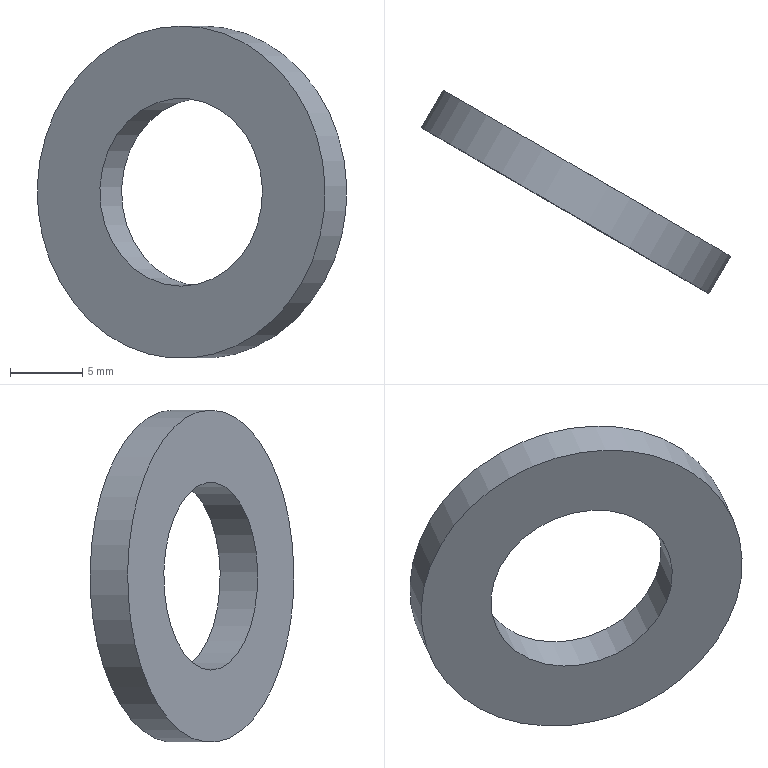Component | NX | WASHER13 | 1 solid | 4 faces | box 21.42 x 14.1 x 23 mm | volume 848 mm3 | cylinder 2 | plane 2 | commonest cylinder face diameters 23 x1 13 x1
STEP:
#1=CARTESIAN_POINT('',(0.,0.,0.));
#2=DIRECTION('',(0.,0.,1.));
#3=DIRECTION('',(1.,0.,0.));
#4=AXIS2_PLACEMENT_3D('',#1,#2,#3);
#5=CARTESIAN_POINT('',(140.906,-62.877,-48.035));
#6=VERTEX_POINT('',#5);
#7=CARTESIAN_POINT('',(137.904,-61.144,-59.));
#8=DIRECTION('',(-0.5,-0.866,0.));
#9=DIRECTION('',(0.2611,-0.1507,0.9535));
#10=AXIS2_PLACEMENT_3D('',#7,#8,#9);
#11=CIRCLE('',#10,11.5);
#12=CARTESIAN_POINT('',(137.904,-61.144,-59.));
#13=DIRECTION('',(0.5,0.866,0.));
#14=DIRECTION('',(-0.2611,0.1507,-0.9535));
#15=AXIS2_PLACEMENT_3D('',#12,#13,#14);
#16=CYLINDRICAL_SURFACE('',#15,11.5);
#17=CARTESIAN_POINT('',(9.425,0.));
#18=DIRECTION('',(-1.,0.));
#19=VECTOR('',#18,1.);
#20=LINE('',#17,#19);
#21=(GEOMETRIC_REPRESENTATION_CONTEXT(2)PARAMETRIC_REPRESENTATION_CONTEXT()REPRESENTATION_CONTEXT('',''));
#22=DEFINITIONAL_REPRESENTATION('',(#20),#21);
#23=PCURVE('',#16,#22);
#24=CARTESIAN_POINT('',(137.904,-61.144,-59.));
#25=DIRECTION('',(-0.5,-0.866,0.));
#26=DIRECTION('',(0.2611,-0.1507,0.9535));
#27=AXIS2_PLACEMENT_3D('',#24,#25,#26);
#28=PLANE('',#27);
#29=CARTESIAN_POINT('',(0.,0.));
#30=DIRECTION('',(1.,0.));
#31=AXIS2_PLACEMENT_2D('',#29,#30);
#32=CIRCLE('',#31,11.5);
#33=(GEOMETRIC_REPRESENTATION_CONTEXT(2)PARAMETRIC_REPRESENTATION_CONTEXT()REPRESENTATION_CONTEXT('',''));
#34=DEFINITIONAL_REPRESENTATION('',(#32),#33);
#35=PCURVE('',#28,#34);
#36=SURFACE_CURVE('',#11,(#23,#35),.PCURVE_S1.);
#37=EDGE_CURVE('',#6,#6,#36,.T.);
#38=ORIENTED_EDGE('',*,*,#37,.F.);
#39=CARTESIAN_POINT('',(142.406,-60.279,-48.035));
#40=VERTEX_POINT('',#39);
#41=CARTESIAN_POINT('',(140.906,-62.877,-48.035));
#42=CARTESIAN_POINT('',(142.406,-60.279,-48.035));
#43=B_SPLINE_CURVE_WITH_KNOTS('',1,(#41,#42),.UNSPECIFIED.,.F.,.F.,(2,2),(0.,3.),.PIECEWISE_BEZIER_KNOTS.);
#44=CARTESIAN_POINT('',(9.425,0.));
#45=DIRECTION('',(0.,1.));
#46=VECTOR('',#45,1.);
#47=LINE('',#44,#46);
#48=(GEOMETRIC_REPRESENTATION_CONTEXT(2)PARAMETRIC_REPRESENTATION_CONTEXT()REPRESENTATION_CONTEXT('',''));
#49=DEFINITIONAL_REPRESENTATION('',(#47),#48);
#50=PCURVE('',#16,#49);
#51=CARTESIAN_POINT('',(3.142,0.));
#52=DIRECTION('',(0.,1.));
#53=VECTOR('',#52,1.);
#54=LINE('',#51,#53);
#55=(GEOMETRIC_REPRESENTATION_CONTEXT(2)PARAMETRIC_REPRESENTATION_CONTEXT()REPRESENTATION_CONTEXT('',''));
#56=DEFINITIONAL_REPRESENTATION('',(#54),#55);
#57=PCURVE('',#16,#56);
#58=SEAM_CURVE('',#43,(#50,#57),.PCURVE_S1.);
#59=EDGE_CURVE('',#6,#40,#58,.T.);
#60=ORIENTED_EDGE('',*,*,#59,.T.);
#61=CARTESIAN_POINT('',(139.404,-58.546,-59.));
#62=DIRECTION('',(-0.5,-0.866,0.));
#63=DIRECTION('',(0.2611,-0.1507,0.9535));
#64=AXIS2_PLACEMENT_3D('',#61,#62,#63);
#65=CIRCLE('',#64,11.5);
#66=CARTESIAN_POINT('',(9.425,3.));
#67=DIRECTION('',(-1.,0.));
#68=VECTOR('',#67,1.);
#69=LINE('',#66,#68);
#70=(GEOMETRIC_REPRESENTATION_CONTEXT(2)PARAMETRIC_REPRESENTATION_CONTEXT()REPRESENTATION_CONTEXT('',''));
#71=DEFINITIONAL_REPRESENTATION('',(#69),#70);
#72=PCURVE('',#16,#71);
#73=CARTESIAN_POINT('',(139.404,-58.546,-59.));
#74=DIRECTION('',(-0.5,-0.866,0.));
#75=DIRECTION('',(0.2611,-0.1507,0.9535));
#76=AXIS2_PLACEMENT_3D('',#73,#74,#75);
#77=PLANE('',#76);
#78=CARTESIAN_POINT('',(0.,0.));
#79=DIRECTION('',(1.,0.));
#80=AXIS2_PLACEMENT_2D('',#78,#79);
#81=CIRCLE('',#80,11.5);
#82=(GEOMETRIC_REPRESENTATION_CONTEXT(2)PARAMETRIC_REPRESENTATION_CONTEXT()REPRESENTATION_CONTEXT('',''));
#83=DEFINITIONAL_REPRESENTATION('',(#81),#82);
#84=PCURVE('',#77,#83);
#85=SURFACE_CURVE('',#65,(#72,#84),.PCURVE_S1.);
#86=EDGE_CURVE('',#40,#40,#85,.T.);
#87=ORIENTED_EDGE('',*,*,#86,.T.);
#88=ORIENTED_EDGE('',*,*,#59,.F.);
#89=EDGE_LOOP('',(#38,#60,#87,#88));
#90=FACE_BOUND('',#89,.T.);
#91=ADVANCED_FACE('',(#90),#16,.T.);
#92=CARTESIAN_POINT('',(139.601,-62.123,-52.802));
#93=VERTEX_POINT('',#92);
#94=CARTESIAN_POINT('',(137.904,-61.144,-59.));
#95=DIRECTION('',(-0.5,-0.866,0.));
#96=DIRECTION('',(0.2611,-0.1507,0.9535));
#97=AXIS2_PLACEMENT_3D('',#94,#95,#96);
#98=CIRCLE('',#97,6.5);
#99=CARTESIAN_POINT('',(137.904,-61.144,-59.));
#100=DIRECTION('',(0.5,0.866,0.));
#101=DIRECTION('',(-0.2611,0.1507,-0.9535));
#102=AXIS2_PLACEMENT_3D('',#99,#100,#101);
#103=CYLINDRICAL_SURFACE('',#102,6.5);
#104=CARTESIAN_POINT('',(9.425,-0.));
#105=DIRECTION('',(-1.,0.));
#106=VECTOR('',#105,1.);
#107=LINE('',#104,#106);
#108=(GEOMETRIC_REPRESENTATION_CONTEXT(2)PARAMETRIC_REPRESENTATION_CONTEXT()REPRESENTATION_CONTEXT('',''));
#109=DEFINITIONAL_REPRESENTATION('',(#107),#108);
#110=PCURVE('',#103,#109);
#111=CARTESIAN_POINT('',(0.,0.));
#112=DIRECTION('',(1.,0.));
#113=AXIS2_PLACEMENT_2D('',#111,#112);
#114=CIRCLE('',#113,6.5);
#115=(GEOMETRIC_REPRESENTATION_CONTEXT(2)PARAMETRIC_REPRESENTATION_CONTEXT()REPRESENTATION_CONTEXT('',''));
#116=DEFINITIONAL_REPRESENTATION('',(#114),#115);
#117=PCURVE('',#28,#116);
#118=SURFACE_CURVE('',#98,(#110,#117),.PCURVE_S1.);
#119=EDGE_CURVE('',#93,#93,#118,.T.);
#120=ORIENTED_EDGE('',*,*,#119,.F.);
#121=CARTESIAN_POINT('',(141.101,-59.525,-52.802));
#122=VERTEX_POINT('',#121);
#123=CARTESIAN_POINT('',(139.601,-62.123,-52.802));
#124=CARTESIAN_POINT('',(141.101,-59.525,-52.802));
#125=B_SPLINE_CURVE_WITH_KNOTS('',1,(#123,#124),.UNSPECIFIED.,.F.,.F.,(2,2),(-0.,3.),.PIECEWISE_BEZIER_KNOTS.);
#126=CARTESIAN_POINT('',(9.425,0.));
#127=DIRECTION('',(0.,1.));
#128=VECTOR('',#127,1.);
#129=LINE('',#126,#128);
#130=(GEOMETRIC_REPRESENTATION_CONTEXT(2)PARAMETRIC_REPRESENTATION_CONTEXT()REPRESENTATION_CONTEXT('',''));
#131=DEFINITIONAL_REPRESENTATION('',(#129),#130);
#132=PCURVE('',#103,#131);
#133=CARTESIAN_POINT('',(3.142,0.));
#134=DIRECTION('',(0.,1.));
#135=VECTOR('',#134,1.);
#136=LINE('',#133,#135);
#137=(GEOMETRIC_REPRESENTATION_CONTEXT(2)PARAMETRIC_REPRESENTATION_CONTEXT()REPRESENTATION_CONTEXT('',''));
#138=DEFINITIONAL_REPRESENTATION('',(#136),#137);
#139=PCURVE('',#103,#138);
#140=SEAM_CURVE('',#125,(#132,#139),.PCURVE_S1.);
#141=EDGE_CURVE('',#93,#122,#140,.T.);
#142=ORIENTED_EDGE('',*,*,#141,.T.);
#143=CARTESIAN_POINT('',(139.404,-58.546,-59.));
#144=DIRECTION('',(-0.5,-0.866,0.));
#145=DIRECTION('',(0.2611,-0.1507,0.9535));
#146=AXIS2_PLACEMENT_3D('',#143,#144,#145);
#147=CIRCLE('',#146,6.5);
#148=CARTESIAN_POINT('',(9.425,3.));
#149=DIRECTION('',(-1.,0.));
#150=VECTOR('',#149,1.);
#151=LINE('',#148,#150);
#152=(GEOMETRIC_REPRESENTATION_CONTEXT(2)PARAMETRIC_REPRESENTATION_CONTEXT()REPRESENTATION_CONTEXT('',''));
#153=DEFINITIONAL_REPRESENTATION('',(#151),#152);
#154=PCURVE('',#103,#153);
#155=CARTESIAN_POINT('',(0.,0.));
#156=DIRECTION('',(1.,0.));
#157=AXIS2_PLACEMENT_2D('',#155,#156);
#158=CIRCLE('',#157,6.5);
#159=(GEOMETRIC_REPRESENTATION_CONTEXT(2)PARAMETRIC_REPRESENTATION_CONTEXT()REPRESENTATION_CONTEXT('',''));
#160=DEFINITIONAL_REPRESENTATION('',(#158),#159);
#161=PCURVE('',#77,#160);
#162=SURFACE_CURVE('',#147,(#154,#161),.PCURVE_S1.);
#163=EDGE_CURVE('',#122,#122,#162,.T.);
#164=ORIENTED_EDGE('',*,*,#163,.T.);
#165=ORIENTED_EDGE('',*,*,#141,.F.);
#166=EDGE_LOOP('',(#120,#142,#164,#165));
#167=FACE_BOUND('',#166,.F.);
#168=ADVANCED_FACE('',(#167),#103,.F.);
#169=ORIENTED_EDGE('',*,*,#37,.T.);
#170=EDGE_LOOP('',(#169));
#171=FACE_BOUND('',#170,.T.);
#172=ORIENTED_EDGE('',*,*,#119,.F.);
#173=EDGE_LOOP('',(#172));
#174=FACE_BOUND('',#173,.T.);
#175=ADVANCED_FACE('',(#171,#174),#28,.T.);
#176=ORIENTED_EDGE('',*,*,#86,.F.);
#177=EDGE_LOOP('',(#176));
#178=FACE_BOUND('',#177,.T.);
#179=ORIENTED_EDGE('',*,*,#163,.T.);
#180=EDGE_LOOP('',(#179));
#181=FACE_BOUND('',#180,.T.);
#182=ADVANCED_FACE('',(#178,#181),#77,.F.);
#183=CLOSED_SHELL('',(#91,#168,#175,#182));
#184=MANIFOLD_SOLID_BREP('',#183);
#185=(LENGTH_UNIT()NAMED_UNIT(*)SI_UNIT(.MILLI.,.METRE.));
#186=UNCERTAINTY_MEASURE_WITH_UNIT(LENGTH_MEASURE(0.00001),#185,'','');
#187=(NAMED_UNIT(*)PLANE_ANGLE_UNIT()SI_UNIT($,.RADIAN.));
#188=(NAMED_UNIT(*)SI_UNIT($,.STERADIAN.)SOLID_ANGLE_UNIT());
#189=(GEOMETRIC_REPRESENTATION_CONTEXT(3)GLOBAL_UNCERTAINTY_ASSIGNED_CONTEXT((#186))GLOBAL_UNIT_ASSIGNED_CONTEXT((#185,#187,#188))REPRESENTATION_CONTEXT('',''));
#190=ADVANCED_BREP_SHAPE_REPRESENTATION('',(#4,#184),#189);